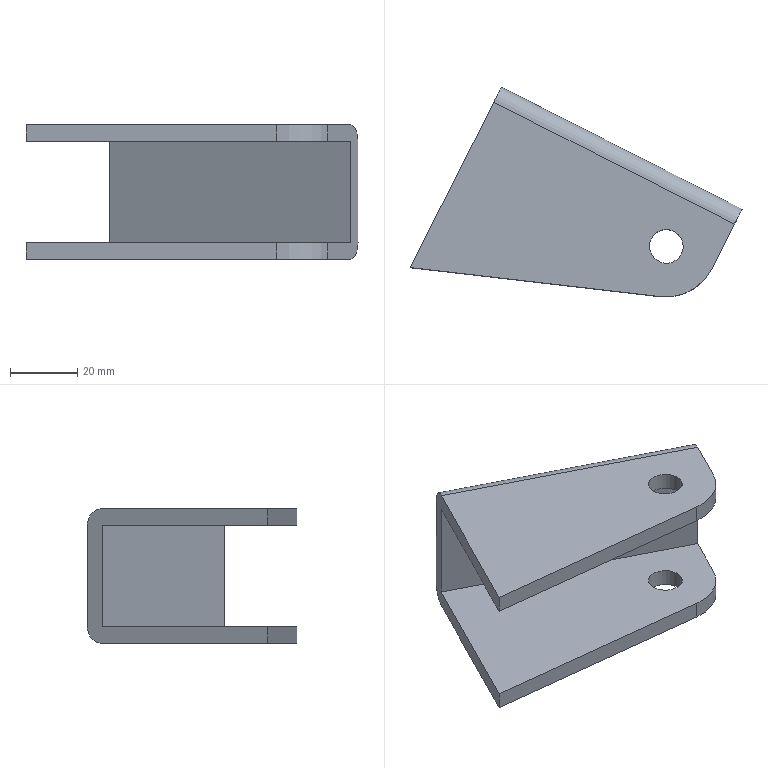Component | SolidWorks | AdjustmentEarPlate-1 | 1 solid | 18 faces | box 98.48 x 62.23 x 40 mm | volume 46338 mm3 | plane 10 | cylinder 8 | commonest cylinder face diameters 10 x6 30 x2
STEP:
#1=CARTESIAN_POINT('',(15.11,-44.59,70.786));
#2=VERTEX_POINT('',#1);
#3=CARTESIAN_POINT('',(14.759,-44.412,70.786));
#4=VERTEX_POINT('',#3);
#5=CARTESIAN_POINT('',(14.934,-44.501,70.786));
#6=DIRECTION('',(0.,0.,-1.));
#7=DIRECTION('',(-0.892,0.4521,0.));
#8=AXIS2_PLACEMENT_3D('',#5,#6,#7);
#9=CIRCLE('',#8,0.1969);
#10=EDGE_CURVE('',#2,#4,#9,.T.);
#11=ORIENTED_EDGE('',*,*,#10,.F.);
#12=CARTESIAN_POINT('',(15.11,-44.59,70.589));
#13=VERTEX_POINT('',#12);
#14=CARTESIAN_POINT('',(15.11,-44.59,72.164));
#15=DIRECTION('',(0.,0.,-1.));
#16=VECTOR('',#15,39.37);
#17=LINE('',#14,#16);
#18=EDGE_CURVE('',#2,#13,#17,.T.);
#19=ORIENTED_EDGE('',*,*,#18,.T.);
#20=CARTESIAN_POINT('',(14.759,-44.412,70.589));
#21=VERTEX_POINT('',#20);
#22=CARTESIAN_POINT('',(14.934,-44.501,70.589));
#23=DIRECTION('',(0.,0.,-1.));
#24=DIRECTION('',(-0.892,0.4521,0.));
#25=AXIS2_PLACEMENT_3D('',#22,#23,#24);
#26=CIRCLE('',#25,0.1969);
#27=EDGE_CURVE('',#13,#21,#26,.T.);
#28=ORIENTED_EDGE('',*,*,#27,.T.);
#29=CARTESIAN_POINT('',(14.759,-44.412,72.164));
#30=DIRECTION('',(0.,0.,-1.));
#31=VECTOR('',#30,39.37);
#32=LINE('',#29,#31);
#33=EDGE_CURVE('',#4,#21,#32,.T.);
#34=ORIENTED_EDGE('',*,*,#33,.F.);
#35=EDGE_LOOP('',(#11,#19,#28,#34));
#36=FACE_OUTER_BOUND('',#35,.T.);
#37=CARTESIAN_POINT('',(14.934,-44.501,72.164));
#38=DIRECTION('',(0.,0.,-1.));
#39=DIRECTION('',(-0.892,0.4521,0.));
#40=AXIS2_PLACEMENT_3D('',#37,#38,#39);
#41=CYLINDRICAL_SURFACE('',#40,0.1969);
#42=ADVANCED_FACE('',(#36),#41,.F.);
#43=CARTESIAN_POINT('',(15.11,-44.59,72.164));
#44=VERTEX_POINT('',#43);
#45=CARTESIAN_POINT('',(14.759,-44.412,72.164));
#46=VERTEX_POINT('',#45);
#47=CARTESIAN_POINT('',(14.934,-44.501,72.164));
#48=DIRECTION('',(0.,0.,-1.));
#49=DIRECTION('',(-0.892,0.4521,0.));
#50=AXIS2_PLACEMENT_3D('',#47,#48,#49);
#51=CIRCLE('',#50,0.1969);
#52=EDGE_CURVE('',#44,#46,#51,.T.);
#53=ORIENTED_EDGE('',*,*,#52,.F.);
#54=CARTESIAN_POINT('',(15.11,-44.59,71.967));
#55=VERTEX_POINT('',#54);
#56=CARTESIAN_POINT('',(15.11,-44.59,72.164));
#57=DIRECTION('',(0.,0.,-1.));
#58=VECTOR('',#57,39.37);
#59=LINE('',#56,#58);
#60=EDGE_CURVE('',#44,#55,#59,.T.);
#61=ORIENTED_EDGE('',*,*,#60,.T.);
#62=CARTESIAN_POINT('',(14.759,-44.412,71.967));
#63=VERTEX_POINT('',#62);
#64=CARTESIAN_POINT('',(14.934,-44.501,71.967));
#65=DIRECTION('',(0.,0.,-1.));
#66=DIRECTION('',(-0.892,0.4521,0.));
#67=AXIS2_PLACEMENT_3D('',#64,#65,#66);
#68=CIRCLE('',#67,0.1969);
#69=EDGE_CURVE('',#55,#63,#68,.T.);
#70=ORIENTED_EDGE('',*,*,#69,.T.);
#71=CARTESIAN_POINT('',(14.759,-44.412,72.164));
#72=DIRECTION('',(0.,0.,-1.));
#73=VECTOR('',#72,39.37);
#74=LINE('',#71,#73);
#75=EDGE_CURVE('',#46,#63,#74,.T.);
#76=ORIENTED_EDGE('',*,*,#75,.F.);
#77=EDGE_LOOP('',(#53,#61,#70,#76));
#78=FACE_OUTER_BOUND('',#77,.T.);
#79=CARTESIAN_POINT('',(14.934,-44.501,72.164));
#80=DIRECTION('',(0.,0.,-1.));
#81=DIRECTION('',(-0.892,0.4521,0.));
#82=AXIS2_PLACEMENT_3D('',#79,#80,#81);
#83=CYLINDRICAL_SURFACE('',#82,0.1969);
#84=ADVANCED_FACE('',(#78),#83,.F.);
#85=CARTESIAN_POINT('',(15.461,-44.767,71.967));
#86=VERTEX_POINT('',#85);
#87=CARTESIAN_POINT('',(14.866,-45.087,71.967));
#88=VERTEX_POINT('',#87);
#89=CARTESIAN_POINT('',(14.934,-44.501,71.967));
#90=DIRECTION('',(0.,0.,-1.));
#91=DIRECTION('',(-0.892,0.4521,0.));
#92=AXIS2_PLACEMENT_3D('',#89,#90,#91);
#93=CIRCLE('',#92,0.5906);
#94=EDGE_CURVE('',#86,#88,#93,.T.);
#95=ORIENTED_EDGE('',*,*,#94,.F.);
#96=CARTESIAN_POINT('',(15.461,-44.767,72.164));
#97=VERTEX_POINT('',#96);
#98=CARTESIAN_POINT('',(15.461,-44.767,70.589));
#99=DIRECTION('',(-0.,-0.,1.));
#100=VECTOR('',#99,39.37);
#101=LINE('',#98,#100);
#102=EDGE_CURVE('',#86,#97,#101,.T.);
#103=ORIENTED_EDGE('',*,*,#102,.T.);
#104=CARTESIAN_POINT('',(14.866,-45.087,72.164));
#105=VERTEX_POINT('',#104);
#106=CARTESIAN_POINT('',(14.934,-44.501,72.164));
#107=DIRECTION('',(0.,0.,-1.));
#108=DIRECTION('',(-0.892,0.4521,0.));
#109=AXIS2_PLACEMENT_3D('',#106,#107,#108);
#110=CIRCLE('',#109,0.5906);
#111=EDGE_CURVE('',#97,#105,#110,.T.);
#112=ORIENTED_EDGE('',*,*,#111,.T.);
#113=CARTESIAN_POINT('',(14.866,-45.087,70.589));
#114=DIRECTION('',(-0.,-0.,1.));
#115=VECTOR('',#114,39.37);
#116=LINE('',#113,#115);
#117=EDGE_CURVE('',#88,#105,#116,.T.);
#118=ORIENTED_EDGE('',*,*,#117,.F.);
#119=EDGE_LOOP('',(#95,#103,#112,#118));
#120=FACE_OUTER_BOUND('',#119,.T.);
#121=CARTESIAN_POINT('',(14.934,-44.501,70.589));
#122=DIRECTION('',(-0.,-0.,1.));
#123=DIRECTION('',(0.892,-0.4521,-0.));
#124=AXIS2_PLACEMENT_3D('',#121,#122,#123);
#125=CYLINDRICAL_SURFACE('',#124,0.5906);
#126=ADVANCED_FACE('',(#120),#125,.T.);
#127=CARTESIAN_POINT('',(11.94,-44.748,71.967));
#128=VERTEX_POINT('',#127);
#129=CARTESIAN_POINT('',(11.94,-44.748,71.967));
#130=DIRECTION('',(-0.9934,0.115,-0.));
#131=VECTOR('',#130,39.37);
#132=LINE('',#129,#131);
#133=EDGE_CURVE('',#88,#128,#132,.T.);
#134=ORIENTED_EDGE('',*,*,#133,.F.);
#135=ORIENTED_EDGE('',*,*,#117,.T.);
#136=CARTESIAN_POINT('',(11.94,-44.748,72.164));
#137=VERTEX_POINT('',#136);
#138=CARTESIAN_POINT('',(11.94,-44.748,72.164));
#139=DIRECTION('',(-0.9934,0.115,-0.));
#140=VECTOR('',#139,39.37);
#141=LINE('',#138,#140);
#142=EDGE_CURVE('',#105,#137,#141,.T.);
#143=ORIENTED_EDGE('',*,*,#142,.T.);
#144=CARTESIAN_POINT('',(11.94,-44.748,70.589));
#145=DIRECTION('',(-0.,-0.,1.));
#146=VECTOR('',#145,39.37);
#147=LINE('',#144,#146);
#148=EDGE_CURVE('',#128,#137,#147,.T.);
#149=ORIENTED_EDGE('',*,*,#148,.F.);
#150=EDGE_LOOP('',(#134,#135,#143,#149));
#151=FACE_OUTER_BOUND('',#150,.T.);
#152=CARTESIAN_POINT('',(11.94,-44.748,70.589));
#153=DIRECTION('',(0.115,0.9934,0.));
#154=DIRECTION('',(0.9934,-0.115,0.));
#155=AXIS2_PLACEMENT_3D('',#152,#153,#154);
#156=PLANE('',#155);
#157=ADVANCED_FACE('',(#151),#156,.F.);
#158=CARTESIAN_POINT('',(12.918,-42.817,72.164));
#159=VERTEX_POINT('',#158);
#160=CARTESIAN_POINT('',(13.007,-42.641,72.164));
#161=DIRECTION('',(0.4521,0.892,0.));
#162=VECTOR('',#161,39.37);
#163=LINE('',#160,#162);
#164=EDGE_CURVE('',#137,#159,#163,.T.);
#165=ORIENTED_EDGE('',*,*,#164,.T.);
#166=CARTESIAN_POINT('',(13.007,-42.641,71.967));
#167=VERTEX_POINT('',#166);
#168=CARTESIAN_POINT('',(12.918,-42.817,71.967));
#169=DIRECTION('',(-0.892,0.4521,0.));
#170=DIRECTION('',(-0.4521,-0.892,-0.));
#171=AXIS2_PLACEMENT_3D('',#168,#169,#170);
#172=CIRCLE('',#171,0.1969);
#173=EDGE_CURVE('',#159,#167,#172,.T.);
#174=ORIENTED_EDGE('',*,*,#173,.T.);
#175=CARTESIAN_POINT('',(13.007,-42.641,70.786));
#176=VERTEX_POINT('',#175);
#177=CARTESIAN_POINT('',(13.007,-42.641,70.589));
#178=DIRECTION('',(-0.,-0.,1.));
#179=VECTOR('',#178,39.37);
#180=LINE('',#177,#179);
#181=EDGE_CURVE('',#176,#167,#180,.T.);
#182=ORIENTED_EDGE('',*,*,#181,.F.);
#183=CARTESIAN_POINT('',(12.918,-42.817,70.589));
#184=VERTEX_POINT('',#183);
#185=CARTESIAN_POINT('',(12.918,-42.817,70.786));
#186=DIRECTION('',(-0.892,0.4521,0.));
#187=DIRECTION('',(-0.4521,-0.892,-0.));
#188=AXIS2_PLACEMENT_3D('',#185,#186,#187);
#189=CIRCLE('',#188,0.1969);
#190=EDGE_CURVE('',#176,#184,#189,.T.);
#191=ORIENTED_EDGE('',*,*,#190,.T.);
#192=CARTESIAN_POINT('',(11.94,-44.748,70.589));
#193=VERTEX_POINT('',#192);
#194=CARTESIAN_POINT('',(13.007,-42.641,70.589));
#195=DIRECTION('',(0.4521,0.892,0.));
#196=VECTOR('',#195,39.37);
#197=LINE('',#194,#196);
#198=EDGE_CURVE('',#193,#184,#197,.T.);
#199=ORIENTED_EDGE('',*,*,#198,.F.);
#200=CARTESIAN_POINT('',(11.94,-44.748,70.786));
#201=VERTEX_POINT('',#200);
#202=CARTESIAN_POINT('',(11.94,-44.748,70.589));
#203=DIRECTION('',(-0.,-0.,1.));
#204=VECTOR('',#203,39.37);
#205=LINE('',#202,#204);
#206=EDGE_CURVE('',#193,#201,#205,.T.);
#207=ORIENTED_EDGE('',*,*,#206,.T.);
#208=CARTESIAN_POINT('',(12.918,-42.817,70.786));
#209=VERTEX_POINT('',#208);
#210=CARTESIAN_POINT('',(13.007,-42.641,70.786));
#211=DIRECTION('',(0.4521,0.892,0.));
#212=VECTOR('',#211,39.37);
#213=LINE('',#210,#212);
#214=EDGE_CURVE('',#201,#209,#213,.T.);
#215=ORIENTED_EDGE('',*,*,#214,.T.);
#216=CARTESIAN_POINT('',(12.918,-42.817,71.967));
#217=VERTEX_POINT('',#216);
#218=CARTESIAN_POINT('',(12.918,-42.817,70.589));
#219=DIRECTION('',(-0.,-0.,1.));
#220=VECTOR('',#219,39.37);
#221=LINE('',#218,#220);
#222=EDGE_CURVE('',#209,#217,#221,.T.);
#223=ORIENTED_EDGE('',*,*,#222,.T.);
#224=CARTESIAN_POINT('',(13.007,-42.641,71.967));
#225=DIRECTION('',(0.4521,0.892,0.));
#226=VECTOR('',#225,39.37);
#227=LINE('',#224,#226);
#228=EDGE_CURVE('',#128,#217,#227,.T.);
#229=ORIENTED_EDGE('',*,*,#228,.F.);
#230=ORIENTED_EDGE('',*,*,#148,.T.);
#231=EDGE_LOOP('',(#165,#174,#182,#191,#199,#207,#215,#223,#229,#230));
#232=FACE_OUTER_BOUND('',#231,.T.);
#233=CARTESIAN_POINT('',(13.007,-42.641,70.589));
#234=DIRECTION('',(0.892,-0.4521,-0.));
#235=DIRECTION('',(-0.4521,-0.892,-0.));
#236=AXIS2_PLACEMENT_3D('',#233,#234,#235);
#237=PLANE('',#236);
#238=ADVANCED_FACE('',(#232),#237,.F.);
#239=CARTESIAN_POINT('',(15.817,-44.065,70.786));
#240=VERTEX_POINT('',#239);
#241=CARTESIAN_POINT('',(15.817,-44.065,71.967));
#242=VERTEX_POINT('',#241);
#243=CARTESIAN_POINT('',(15.817,-44.065,70.589));
#244=DIRECTION('',(-0.,-0.,1.));
#245=VECTOR('',#244,39.37);
#246=LINE('',#243,#245);
#247=EDGE_CURVE('',#240,#242,#246,.T.);
#248=ORIENTED_EDGE('',*,*,#247,.T.);
#249=CARTESIAN_POINT('',(15.728,-44.241,72.164));
#250=VERTEX_POINT('',#249);
#251=CARTESIAN_POINT('',(15.728,-44.241,71.967));
#252=DIRECTION('',(0.892,-0.4521,-0.));
#253=DIRECTION('',(0.4521,0.892,0.));
#254=AXIS2_PLACEMENT_3D('',#251,#252,#253);
#255=CIRCLE('',#254,0.1969);
#256=EDGE_CURVE('',#242,#250,#255,.T.);
#257=ORIENTED_EDGE('',*,*,#256,.T.);
#258=CARTESIAN_POINT('',(15.817,-44.065,72.164));
#259=DIRECTION('',(-0.4521,-0.892,-0.));
#260=VECTOR('',#259,39.37);
#261=LINE('',#258,#260);
#262=EDGE_CURVE('',#250,#97,#261,.T.);
#263=ORIENTED_EDGE('',*,*,#262,.T.);
#264=ORIENTED_EDGE('',*,*,#102,.F.);
#265=CARTESIAN_POINT('',(15.728,-44.241,71.967));
#266=VERTEX_POINT('',#265);
#267=CARTESIAN_POINT('',(15.817,-44.065,71.967));
#268=DIRECTION('',(-0.4521,-0.892,-0.));
#269=VECTOR('',#268,39.37);
#270=LINE('',#267,#269);
#271=EDGE_CURVE('',#266,#86,#270,.T.);
#272=ORIENTED_EDGE('',*,*,#271,.F.);
#273=CARTESIAN_POINT('',(15.728,-44.241,70.786));
#274=VERTEX_POINT('',#273);
#275=CARTESIAN_POINT('',(15.728,-44.241,70.589));
#276=DIRECTION('',(-0.,-0.,1.));
#277=VECTOR('',#276,39.37);
#278=LINE('',#275,#277);
#279=EDGE_CURVE('',#274,#266,#278,.T.);
#280=ORIENTED_EDGE('',*,*,#279,.F.);
#281=CARTESIAN_POINT('',(15.461,-44.767,70.786));
#282=VERTEX_POINT('',#281);
#283=CARTESIAN_POINT('',(15.817,-44.065,70.786));
#284=DIRECTION('',(-0.4521,-0.892,-0.));
#285=VECTOR('',#284,39.37);
#286=LINE('',#283,#285);
#287=EDGE_CURVE('',#274,#282,#286,.T.);
#288=ORIENTED_EDGE('',*,*,#287,.T.);
#289=CARTESIAN_POINT('',(15.461,-44.767,70.589));
#290=VERTEX_POINT('',#289);
#291=CARTESIAN_POINT('',(15.461,-44.767,70.589));
#292=DIRECTION('',(-0.,-0.,1.));
#293=VECTOR('',#292,39.37);
#294=LINE('',#291,#293);
#295=EDGE_CURVE('',#290,#282,#294,.T.);
#296=ORIENTED_EDGE('',*,*,#295,.F.);
#297=CARTESIAN_POINT('',(15.728,-44.241,70.589));
#298=VERTEX_POINT('',#297);
#299=CARTESIAN_POINT('',(15.817,-44.065,70.589));
#300=DIRECTION('',(-0.4521,-0.892,-0.));
#301=VECTOR('',#300,39.37);
#302=LINE('',#299,#301);
#303=EDGE_CURVE('',#298,#290,#302,.T.);
#304=ORIENTED_EDGE('',*,*,#303,.F.);
#305=CARTESIAN_POINT('',(15.728,-44.241,70.786));
#306=DIRECTION('',(0.892,-0.4521,-0.));
#307=DIRECTION('',(0.4521,0.892,0.));
#308=AXIS2_PLACEMENT_3D('',#305,#306,#307);
#309=CIRCLE('',#308,0.1969);
#310=EDGE_CURVE('',#298,#240,#309,.T.);
#311=ORIENTED_EDGE('',*,*,#310,.T.);
#312=EDGE_LOOP('',(#248,#257,#263,#264,#272,#280,#288,#296,#304,#311));
#313=FACE_OUTER_BOUND('',#312,.T.);
#314=CARTESIAN_POINT('',(15.817,-44.065,70.589));
#315=DIRECTION('',(-0.892,0.4521,0.));
#316=DIRECTION('',(0.4521,0.892,0.));
#317=AXIS2_PLACEMENT_3D('',#314,#315,#316);
#318=PLANE('',#317);
#319=ADVANCED_FACE('',(#313),#318,.F.);
#320=ORIENTED_EDGE('',*,*,#295,.T.);
#321=CARTESIAN_POINT('',(14.866,-45.087,70.786));
#322=VERTEX_POINT('',#321);
#323=CARTESIAN_POINT('',(14.934,-44.501,70.786));
#324=DIRECTION('',(0.,0.,-1.));
#325=DIRECTION('',(-0.892,0.4521,0.));
#326=AXIS2_PLACEMENT_3D('',#323,#324,#325);
#327=CIRCLE('',#326,0.5906);
#328=EDGE_CURVE('',#282,#322,#327,.T.);
#329=ORIENTED_EDGE('',*,*,#328,.T.);
#330=CARTESIAN_POINT('',(14.866,-45.087,70.589));
#331=VERTEX_POINT('',#330);
#332=CARTESIAN_POINT('',(14.866,-45.087,70.589));
#333=DIRECTION('',(-0.,-0.,1.));
#334=VECTOR('',#333,39.37);
#335=LINE('',#332,#334);
#336=EDGE_CURVE('',#331,#322,#335,.T.);
#337=ORIENTED_EDGE('',*,*,#336,.F.);
#338=CARTESIAN_POINT('',(14.934,-44.501,70.589));
#339=DIRECTION('',(0.,0.,-1.));
#340=DIRECTION('',(-0.892,0.4521,0.));
#341=AXIS2_PLACEMENT_3D('',#338,#339,#340);
#342=CIRCLE('',#341,0.5906);
#343=EDGE_CURVE('',#290,#331,#342,.T.);
#344=ORIENTED_EDGE('',*,*,#343,.F.);
#345=EDGE_LOOP('',(#320,#329,#337,#344));
#346=FACE_OUTER_BOUND('',#345,.T.);
#347=CARTESIAN_POINT('',(14.934,-44.501,70.589));
#348=DIRECTION('',(-0.,-0.,1.));
#349=DIRECTION('',(0.892,-0.4521,-0.));
#350=AXIS2_PLACEMENT_3D('',#347,#348,#349);
#351=CYLINDRICAL_SURFACE('',#350,0.5906);
#352=ADVANCED_FACE('',(#346),#351,.T.);
#353=ORIENTED_EDGE('',*,*,#336,.T.);
#354=CARTESIAN_POINT('',(11.94,-44.748,70.786));
#355=DIRECTION('',(-0.9934,0.115,-0.));
#356=VECTOR('',#355,39.37);
#357=LINE('',#354,#356);
#358=EDGE_CURVE('',#322,#201,#357,.T.);
#359=ORIENTED_EDGE('',*,*,#358,.T.);
#360=ORIENTED_EDGE('',*,*,#206,.F.);
#361=CARTESIAN_POINT('',(11.94,-44.748,70.589));
#362=DIRECTION('',(-0.9934,0.115,-0.));
#363=VECTOR('',#362,39.37);
#364=LINE('',#361,#363);
#365=EDGE_CURVE('',#331,#193,#364,.T.);
#366=ORIENTED_EDGE('',*,*,#365,.F.);
#367=EDGE_LOOP('',(#353,#359,#360,#366));
#368=FACE_OUTER_BOUND('',#367,.T.);
#369=CARTESIAN_POINT('',(11.94,-44.748,70.589));
#370=DIRECTION('',(0.115,0.9934,0.));
#371=DIRECTION('',(0.9934,-0.115,0.));
#372=AXIS2_PLACEMENT_3D('',#369,#370,#371);
#373=PLANE('',#372);
#374=ADVANCED_FACE('',(#368),#373,.F.);
#375=ORIENTED_EDGE('',*,*,#181,.T.);
#376=CARTESIAN_POINT('',(15.817,-44.065,71.967));
#377=DIRECTION('',(0.892,-0.4521,-0.));
#378=VECTOR('',#377,39.37);
#379=LINE('',#376,#378);
#380=EDGE_CURVE('',#167,#242,#379,.T.);
#381=ORIENTED_EDGE('',*,*,#380,.T.);
#382=ORIENTED_EDGE('',*,*,#247,.F.);
#383=CARTESIAN_POINT('',(13.007,-42.641,70.786));
#384=DIRECTION('',(-0.892,0.4521,0.));
#385=VECTOR('',#384,39.37);
#386=LINE('',#383,#385);
#387=EDGE_CURVE('',#240,#176,#386,.T.);
#388=ORIENTED_EDGE('',*,*,#387,.T.);
#389=EDGE_LOOP('',(#375,#381,#382,#388));
#390=FACE_OUTER_BOUND('',#389,.T.);
#391=CARTESIAN_POINT('',(15.817,-44.065,70.589));
#392=DIRECTION('',(-0.4521,-0.892,-0.));
#393=DIRECTION('',(-0.892,0.4521,0.));
#394=AXIS2_PLACEMENT_3D('',#391,#392,#393);
#395=PLANE('',#394);
#396=ADVANCED_FACE('',(#390),#395,.F.);
#397=CARTESIAN_POINT('',(14.934,-44.501,70.589));
#398=DIRECTION('',(0.,0.,-1.));
#399=DIRECTION('',(-0.892,0.4521,0.));
#400=AXIS2_PLACEMENT_3D('',#397,#398,#399);
#401=CIRCLE('',#400,0.1969);
#402=EDGE_CURVE('',#21,#13,#401,.T.);
#403=ORIENTED_EDGE('',*,*,#402,.F.);
#404=ORIENTED_EDGE('',*,*,#27,.F.);
#405=EDGE_LOOP('',(#403,#404));
#406=FACE_BOUND('',#405,.T.);
#407=ORIENTED_EDGE('',*,*,#198,.T.);
#408=CARTESIAN_POINT('',(15.728,-44.241,70.589));
#409=DIRECTION('',(0.892,-0.4521,-0.));
#410=VECTOR('',#409,39.37);
#411=LINE('',#408,#410);
#412=EDGE_CURVE('',#184,#298,#411,.T.);
#413=ORIENTED_EDGE('',*,*,#412,.T.);
#414=ORIENTED_EDGE('',*,*,#303,.T.);
#415=ORIENTED_EDGE('',*,*,#343,.T.);
#416=ORIENTED_EDGE('',*,*,#365,.T.);
#417=EDGE_LOOP('',(#407,#413,#414,#415,#416));
#418=FACE_OUTER_BOUND('',#417,.T.);
#419=CARTESIAN_POINT('',(14.934,-44.501,70.589));
#420=DIRECTION('',(0.,0.,-1.));
#421=DIRECTION('',(-0.892,0.4521,0.));
#422=AXIS2_PLACEMENT_3D('',#419,#420,#421);
#423=PLANE('',#422);
#424=ADVANCED_FACE('',(#406,#418),#423,.T.);
#425=CARTESIAN_POINT('',(14.934,-44.501,72.164));
#426=DIRECTION('',(0.,0.,-1.));
#427=DIRECTION('',(-0.892,0.4521,0.));
#428=AXIS2_PLACEMENT_3D('',#425,#426,#427);
#429=CIRCLE('',#428,0.1969);
#430=EDGE_CURVE('',#46,#44,#429,.T.);
#431=ORIENTED_EDGE('',*,*,#430,.T.);
#432=ORIENTED_EDGE('',*,*,#52,.T.);
#433=EDGE_LOOP('',(#431,#432));
#434=FACE_BOUND('',#433,.T.);
#435=ORIENTED_EDGE('',*,*,#262,.F.);
#436=CARTESIAN_POINT('',(15.201,-43.974,72.164));
#437=DIRECTION('',(-0.892,0.4521,0.));
#438=VECTOR('',#437,39.37);
#439=LINE('',#436,#438);
#440=EDGE_CURVE('',#250,#159,#439,.T.);
#441=ORIENTED_EDGE('',*,*,#440,.T.);
#442=ORIENTED_EDGE('',*,*,#164,.F.);
#443=ORIENTED_EDGE('',*,*,#142,.F.);
#444=ORIENTED_EDGE('',*,*,#111,.F.);
#445=EDGE_LOOP('',(#435,#441,#442,#443,#444));
#446=FACE_OUTER_BOUND('',#445,.T.);
#447=CARTESIAN_POINT('',(14.934,-44.501,72.164));
#448=DIRECTION('',(0.,0.,-1.));
#449=DIRECTION('',(-0.892,0.4521,0.));
#450=AXIS2_PLACEMENT_3D('',#447,#448,#449);
#451=PLANE('',#450);
#452=ADVANCED_FACE('',(#434,#446),#451,.F.);
#453=CARTESIAN_POINT('',(15.728,-44.241,71.967));
#454=DIRECTION('',(0.892,-0.4521,-0.));
#455=VECTOR('',#454,39.37);
#456=LINE('',#453,#455);
#457=EDGE_CURVE('',#217,#266,#456,.T.);
#458=ORIENTED_EDGE('',*,*,#457,.F.);
#459=ORIENTED_EDGE('',*,*,#222,.F.);
#460=CARTESIAN_POINT('',(15.728,-44.241,70.786));
#461=DIRECTION('',(0.892,-0.4521,-0.));
#462=VECTOR('',#461,39.37);
#463=LINE('',#460,#462);
#464=EDGE_CURVE('',#209,#274,#463,.T.);
#465=ORIENTED_EDGE('',*,*,#464,.T.);
#466=ORIENTED_EDGE('',*,*,#279,.T.);
#467=EDGE_LOOP('',(#458,#459,#465,#466));
#468=FACE_OUTER_BOUND('',#467,.T.);
#469=CARTESIAN_POINT('',(15.728,-44.241,70.589));
#470=DIRECTION('',(-0.4521,-0.892,-0.));
#471=DIRECTION('',(-0.892,0.4521,0.));
#472=AXIS2_PLACEMENT_3D('',#469,#470,#471);
#473=PLANE('',#472);
#474=ADVANCED_FACE('',(#468),#473,.T.);
#475=CARTESIAN_POINT('',(14.934,-44.501,70.786));
#476=DIRECTION('',(0.,0.,-1.));
#477=DIRECTION('',(-0.892,0.4521,0.));
#478=AXIS2_PLACEMENT_3D('',#475,#476,#477);
#479=CIRCLE('',#478,0.1969);
#480=EDGE_CURVE('',#4,#2,#479,.T.);
#481=ORIENTED_EDGE('',*,*,#480,.T.);
#482=ORIENTED_EDGE('',*,*,#10,.T.);
#483=EDGE_LOOP('',(#481,#482));
#484=FACE_BOUND('',#483,.T.);
#485=ORIENTED_EDGE('',*,*,#328,.F.);
#486=ORIENTED_EDGE('',*,*,#287,.F.);
#487=ORIENTED_EDGE('',*,*,#464,.F.);
#488=ORIENTED_EDGE('',*,*,#214,.F.);
#489=ORIENTED_EDGE('',*,*,#358,.F.);
#490=EDGE_LOOP('',(#485,#486,#487,#488,#489));
#491=FACE_OUTER_BOUND('',#490,.T.);
#492=CARTESIAN_POINT('',(14.934,-44.501,70.786));
#493=DIRECTION('',(0.,0.,-1.));
#494=DIRECTION('',(-0.892,0.4521,0.));
#495=AXIS2_PLACEMENT_3D('',#492,#493,#494);
#496=PLANE('',#495);
#497=ADVANCED_FACE('',(#484,#491),#496,.F.);
#498=CARTESIAN_POINT('',(14.934,-44.501,71.967));
#499=DIRECTION('',(0.,0.,-1.));
#500=DIRECTION('',(-0.892,0.4521,0.));
#501=AXIS2_PLACEMENT_3D('',#498,#499,#500);
#502=CIRCLE('',#501,0.1969);
#503=EDGE_CURVE('',#63,#55,#502,.T.);
#504=ORIENTED_EDGE('',*,*,#503,.F.);
#505=ORIENTED_EDGE('',*,*,#69,.F.);
#506=EDGE_LOOP('',(#504,#505));
#507=FACE_BOUND('',#506,.T.);
#508=ORIENTED_EDGE('',*,*,#94,.T.);
#509=ORIENTED_EDGE('',*,*,#133,.T.);
#510=ORIENTED_EDGE('',*,*,#228,.T.);
#511=ORIENTED_EDGE('',*,*,#457,.T.);
#512=ORIENTED_EDGE('',*,*,#271,.T.);
#513=EDGE_LOOP('',(#508,#509,#510,#511,#512));
#514=FACE_OUTER_BOUND('',#513,.T.);
#515=CARTESIAN_POINT('',(14.934,-44.501,71.967));
#516=DIRECTION('',(0.,0.,-1.));
#517=DIRECTION('',(-0.892,0.4521,0.));
#518=AXIS2_PLACEMENT_3D('',#515,#516,#517);
#519=PLANE('',#518);
#520=ADVANCED_FACE('',(#507,#514),#519,.T.);
#521=ORIENTED_EDGE('',*,*,#60,.F.);
#522=ORIENTED_EDGE('',*,*,#430,.F.);
#523=ORIENTED_EDGE('',*,*,#75,.T.);
#524=ORIENTED_EDGE('',*,*,#503,.T.);
#525=EDGE_LOOP('',(#521,#522,#523,#524));
#526=FACE_OUTER_BOUND('',#525,.T.);
#527=CARTESIAN_POINT('',(14.934,-44.501,72.164));
#528=DIRECTION('',(0.,0.,-1.));
#529=DIRECTION('',(-0.892,0.4521,0.));
#530=AXIS2_PLACEMENT_3D('',#527,#528,#529);
#531=CYLINDRICAL_SURFACE('',#530,0.1969);
#532=ADVANCED_FACE('',(#526),#531,.F.);
#533=ORIENTED_EDGE('',*,*,#18,.F.);
#534=ORIENTED_EDGE('',*,*,#480,.F.);
#535=ORIENTED_EDGE('',*,*,#33,.T.);
#536=ORIENTED_EDGE('',*,*,#402,.T.);
#537=EDGE_LOOP('',(#533,#534,#535,#536));
#538=FACE_OUTER_BOUND('',#537,.T.);
#539=CARTESIAN_POINT('',(14.934,-44.501,72.164));
#540=DIRECTION('',(0.,0.,-1.));
#541=DIRECTION('',(-0.892,0.4521,0.));
#542=AXIS2_PLACEMENT_3D('',#539,#540,#541);
#543=CYLINDRICAL_SURFACE('',#542,0.1969);
#544=ADVANCED_FACE('',(#538),#543,.F.);
#545=ORIENTED_EDGE('',*,*,#173,.F.);
#546=ORIENTED_EDGE('',*,*,#440,.F.);
#547=ORIENTED_EDGE('',*,*,#256,.F.);
#548=ORIENTED_EDGE('',*,*,#380,.F.);
#549=EDGE_LOOP('',(#545,#546,#547,#548));
#550=FACE_OUTER_BOUND('',#549,.T.);
#551=CARTESIAN_POINT('',(15.728,-44.241,71.967));
#552=DIRECTION('',(0.892,-0.4521,-0.));
#553=DIRECTION('',(-0.4521,-0.892,-0.));
#554=AXIS2_PLACEMENT_3D('',#551,#552,#553);
#555=CYLINDRICAL_SURFACE('',#554,0.1969);
#556=ADVANCED_FACE('',(#550),#555,.T.);
#557=ORIENTED_EDGE('',*,*,#190,.F.);
#558=ORIENTED_EDGE('',*,*,#387,.F.);
#559=ORIENTED_EDGE('',*,*,#310,.F.);
#560=ORIENTED_EDGE('',*,*,#412,.F.);
#561=EDGE_LOOP('',(#557,#558,#559,#560));
#562=FACE_OUTER_BOUND('',#561,.T.);
#563=CARTESIAN_POINT('',(15.201,-43.974,70.786));
#564=DIRECTION('',(-0.892,0.4521,0.));
#565=DIRECTION('',(0.4521,0.892,0.));
#566=AXIS2_PLACEMENT_3D('',#563,#564,#565);
#567=CYLINDRICAL_SURFACE('',#566,0.1969);
#568=ADVANCED_FACE('',(#562),#567,.T.);
#569=CLOSED_SHELL('',(#42,#84,#126,#157,#238,#319,#352,#374,#396,#424,#452,#474,#497,#520,#532,#544,#556,#568));
#570=MANIFOLD_SOLID_BREP('',#569);
#571=CARTESIAN_POINT('',(0.,0.,0.));
#572=DIRECTION('',(0.,0.,1.));
#573=DIRECTION('',(1.,0.,0.));
#574=AXIS2_PLACEMENT_3D('',#571,#572,#573);
#575=(LENGTH_UNIT()NAMED_UNIT(*)SI_UNIT($,.METRE.));
#576=LENGTH_MEASURE_WITH_UNIT(LENGTH_MEASURE(0.0254),#575);
#577=DIMENSIONAL_EXPONENTS(1.,0.,0.,0.,0.,0.,0.);
#578=(CONVERSION_BASED_UNIT('',#576)LENGTH_UNIT()NAMED_UNIT(#577));
#579=UNCERTAINTY_MEASURE_WITH_UNIT(LENGTH_MEASURE(0.00001),#578,'','');
#580=(NAMED_UNIT(*)PLANE_ANGLE_UNIT()SI_UNIT($,.RADIAN.));
#581=(NAMED_UNIT(*)SI_UNIT($,.STERADIAN.)SOLID_ANGLE_UNIT());
#582=(GEOMETRIC_REPRESENTATION_CONTEXT(3)GLOBAL_UNCERTAINTY_ASSIGNED_CONTEXT((#579))GLOBAL_UNIT_ASSIGNED_CONTEXT((#578,#580,#581))REPRESENTATION_CONTEXT('',''));
#583=ADVANCED_BREP_SHAPE_REPRESENTATION('',(#570,#574),#582);
#584=COLOUR_RGB('',0.7922,0.8196,0.9333);
#585=FILL_AREA_STYLE_COLOUR('',#584);
#586=FILL_AREA_STYLE('',(#585));
#587=SURFACE_STYLE_FILL_AREA(#586);
#588=SURFACE_SIDE_STYLE('',(#587));
#589=SURFACE_STYLE_USAGE(.BOTH.,#588);
#590=PRESENTATION_STYLE_ASSIGNMENT((#589));
#591=STYLED_ITEM('',(#590),#570);
#592=PRESENTATION_LAYER_ASSIGNMENT('','',(#591));
#593=(LENGTH_UNIT()NAMED_UNIT(*)SI_UNIT($,.METRE.));
#594=LENGTH_MEASURE_WITH_UNIT(LENGTH_MEASURE(0.0254),#593);
#595=DIMENSIONAL_EXPONENTS(1.,0.,0.,0.,0.,0.,0.);
#596=(CONVERSION_BASED_UNIT('',#594)LENGTH_UNIT()NAMED_UNIT(#595));
#597=UNCERTAINTY_MEASURE_WITH_UNIT(LENGTH_MEASURE(0.00001),#596,'','');
#598=(NAMED_UNIT(*)PLANE_ANGLE_UNIT()SI_UNIT($,.RADIAN.));
#599=(NAMED_UNIT(*)SI_UNIT($,.STERADIAN.)SOLID_ANGLE_UNIT());
#600=(GEOMETRIC_REPRESENTATION_CONTEXT(3)GLOBAL_UNCERTAINTY_ASSIGNED_CONTEXT((#597))GLOBAL_UNIT_ASSIGNED_CONTEXT((#596,#598,#599))REPRESENTATION_CONTEXT('',''));
#601=MECHANICAL_DESIGN_GEOMETRIC_PRESENTATION_REPRESENTATION('',(#591),#600);